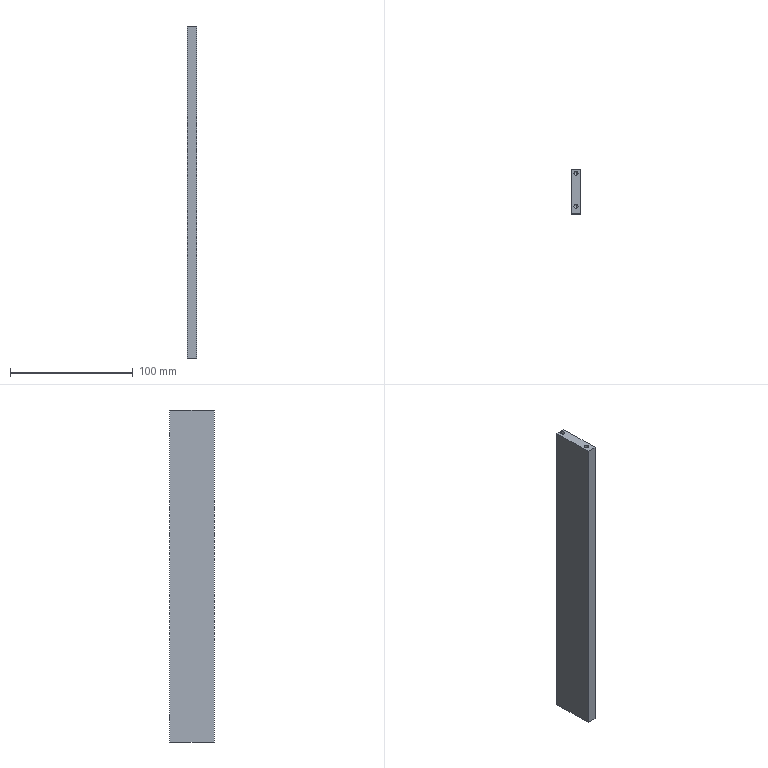Component | SolidWorks | LD101-02--Q1005-Q1-2-2 | 1 solid | 30 faces | box 8 x 36 x 270 mm | volume 77030 mm3 | cylinder 12 | cone 12 | plane 6 | commonest cylinder face diameters 3.3 x12 | material AL6061
build123d program:
from build123d import *

# Parameters (mm, degrees)
SKETCH1_W                  = 270
SKETCH1_H                  = 8
BOSS_EXTRUDE1_DEPTH        = 18
M4_TAPPED_HOLE2_AT_2_COUNT = 2
M4_TAPPED_HOLE2_AT_2_PITCH = 27
M4_TAPPED_HOLE3_D          = 3.3
M4_TAPPED_HOLE3_DEPTH      = 13.5
M4_TAPPED_HOLE3_TIP        = 0.9914


with BuildPart() as part:
    # Sketch1 → Boss-Extrude1 (new, symmetric)
    with BuildSketch(Plane.XY):
        Rectangle(SKETCH1_W, SKETCH1_H)
    extrude(amount=BOSS_EXTRUDE1_DEPTH, both=True)

    # Sketch2 → M4 Tapped Hole2 (revolve, cut)
    with BuildSketch(Plane(origin=(-135, 0, -15), x_dir=(0, 0, 1), z_dir=(0, 1, 0))):
        Polygon((0, 0), (0, 15.091), (1.65, 14.1), (1.65, 0), align=None)
    m4_tapped_hole2 = revolve(axis=Axis((-141.35, 0, -15), (1, 0, 0)), mode=Mode.SUBTRACT)

    # M4 Tapped Hole2 at 2: M4 Tapped Hole2 ×2
    with Locations(*[(0, 0, i * M4_TAPPED_HOLE2_AT_2_PITCH) for i in range(1, M4_TAPPED_HOLE2_AT_2_COUNT)]):
        add(m4_tapped_hole2, mode=Mode.SUBTRACT)

    # Mirror2: M4 Tapped Hole2 across plane
    add(m4_tapped_hole2.mirror(Plane(origin=(0, 0, 0), x_dir=(0, 0, 1), z_dir=(1, 0, 0))), mode=Mode.SUBTRACT)

    # Mirror2 copy 1 sketch → Mirror2 copy 1 (revolve, cut)
    with BuildSketch(Plane(origin=(135, 0, 12), x_dir=(0, 0, 1), z_dir=(0, 1, 0))):
        Polygon((0, 0), (0, -15.091), (1.65, -14.1), (1.65, 0), align=None)
    revolve(axis=Axis((141.35, 0, 12), (1, 0, 0)), mode=Mode.SUBTRACT)

    # M4 Tapped Hole3
    with Locations(Plane(origin=(0, 0, -18), x_dir=(-1, 0, 0), z_dir=(0, 0, -1))):
        with Locations((-115, 0), (115, 0)):
            Hole(M4_TAPPED_HOLE3_D / 2, depth=M4_TAPPED_HOLE3_DEPTH)
            with Locations((0, 0, -(M4_TAPPED_HOLE3_DEPTH + M4_TAPPED_HOLE3_TIP / 2))):  # 118° drill point
                Cone(0, M4_TAPPED_HOLE3_D / 2, M4_TAPPED_HOLE3_TIP, mode=Mode.SUBTRACT)


solid = part.part

# Placed as in the assembly
solid = solid.moved(Location((324.21, -178.897, 146.257), (90, 0, 90)))
STEP:
#1=COLOUR_RGB('',0.7922,0.8196,0.9333);
#2=FILL_AREA_STYLE_COLOUR('',#1);
#3=FILL_AREA_STYLE('',(#2));
#4=SURFACE_STYLE_FILL_AREA(#3);
#5=SURFACE_SIDE_STYLE('',(#4));
#6=SURFACE_STYLE_USAGE(.BOTH.,#5);
#7=PRESENTATION_STYLE_ASSIGNMENT((#6));
#8=CARTESIAN_POINT('',(12.764,-6.866,1.166));
#9=VERTEX_POINT('',#8);
#10=CARTESIAN_POINT('',(12.764,-6.866,1.296));
#11=VERTEX_POINT('',#10);
#12=CARTESIAN_POINT('',(12.764,-6.866,1.231));
#13=DIRECTION('',(0.,1.,0.));
#14=DIRECTION('',(0.,0.,1.));
#15=AXIS2_PLACEMENT_3D('',#12,#13,#14);
#16=CIRCLE('',#15,0.06496);
#17=EDGE_CURVE('',#9,#11,#16,.T.);
#18=ORIENTED_EDGE('',*,*,#17,.F.);
#19=CARTESIAN_POINT('',(12.764,-6.335,1.166));
#20=VERTEX_POINT('',#19);
#21=CARTESIAN_POINT('',(12.764,-6.335,1.166));
#22=DIRECTION('',(0.,1.,0.));
#23=VECTOR('',#22,39.37);
#24=LINE('',#21,#23);
#25=EDGE_CURVE('',#9,#20,#24,.T.);
#26=ORIENTED_EDGE('',*,*,#25,.T.);
#27=CARTESIAN_POINT('',(12.764,-6.335,1.296));
#28=VERTEX_POINT('',#27);
#29=CARTESIAN_POINT('',(12.764,-6.335,1.231));
#30=DIRECTION('',(0.,1.,0.));
#31=DIRECTION('',(0.,0.,1.));
#32=AXIS2_PLACEMENT_3D('',#29,#30,#31);
#33=CIRCLE('',#32,0.06496);
#34=EDGE_CURVE('',#20,#28,#33,.T.);
#35=ORIENTED_EDGE('',*,*,#34,.T.);
#36=CARTESIAN_POINT('',(12.764,-6.335,1.296));
#37=DIRECTION('',(0.,1.,0.));
#38=VECTOR('',#37,39.37);
#39=LINE('',#36,#38);
#40=EDGE_CURVE('',#11,#28,#39,.T.);
#41=ORIENTED_EDGE('',*,*,#40,.F.);
#42=EDGE_LOOP('',(#18,#26,#35,#41));
#43=FACE_OUTER_BOUND('',#42,.T.);
#44=CARTESIAN_POINT('',(12.764,-6.335,1.231));
#45=DIRECTION('',(0.,1.,0.));
#46=DIRECTION('',(0.,0.,1.));
#47=AXIS2_PLACEMENT_3D('',#44,#45,#46);
#48=CYLINDRICAL_SURFACE('',#47,0.06496);
#49=ADVANCED_FACE('',(#43),#48,.F.);
#50=CARTESIAN_POINT('',(12.764,-6.905,1.231));
#51=VERTEX_POINT('',#50);
#52=CARTESIAN_POINT('',(12.764,-6.866,1.296));
#53=DIRECTION('',(-0.,0.515,0.8572));
#54=VECTOR('',#53,39.37);
#55=LINE('',#52,#54);
#56=EDGE_CURVE('',#51,#11,#55,.T.);
#57=ORIENTED_EDGE('',*,*,#56,.F.);
#58=CARTESIAN_POINT('',(12.764,-6.866,1.166));
#59=DIRECTION('',(0.,0.515,-0.8572));
#60=VECTOR('',#59,39.37);
#61=LINE('',#58,#60);
#62=EDGE_CURVE('',#51,#9,#61,.T.);
#63=ORIENTED_EDGE('',*,*,#62,.T.);
#64=ORIENTED_EDGE('',*,*,#17,.T.);
#65=EDGE_LOOP('',(#57,#63,#64));
#66=FACE_OUTER_BOUND('',#65,.T.);
#67=CARTESIAN_POINT('',(12.764,-6.866,1.231));
#68=DIRECTION('',(0.,1.,0.));
#69=DIRECTION('',(0.,0.,1.));
#70=AXIS2_PLACEMENT_3D('',#67,#68,#69);
#71=CONICAL_SURFACE('',#70,0.06496,1.03);
#72=ADVANCED_FACE('',(#66),#71,.F.);
#73=CARTESIAN_POINT('',(12.764,-6.866,10.221));
#74=VERTEX_POINT('',#73);
#75=CARTESIAN_POINT('',(12.764,-6.866,10.351));
#76=VERTEX_POINT('',#75);
#77=CARTESIAN_POINT('',(12.764,-6.866,10.286));
#78=DIRECTION('',(0.,1.,0.));
#79=DIRECTION('',(0.,0.,1.));
#80=AXIS2_PLACEMENT_3D('',#77,#78,#79);
#81=CIRCLE('',#80,0.06496);
#82=EDGE_CURVE('',#74,#76,#81,.T.);
#83=ORIENTED_EDGE('',*,*,#82,.F.);
#84=CARTESIAN_POINT('',(12.764,-6.335,10.221));
#85=VERTEX_POINT('',#84);
#86=CARTESIAN_POINT('',(12.764,-6.335,10.221));
#87=DIRECTION('',(0.,1.,0.));
#88=VECTOR('',#87,39.37);
#89=LINE('',#86,#88);
#90=EDGE_CURVE('',#74,#85,#89,.T.);
#91=ORIENTED_EDGE('',*,*,#90,.T.);
#92=CARTESIAN_POINT('',(12.764,-6.335,10.351));
#93=VERTEX_POINT('',#92);
#94=CARTESIAN_POINT('',(12.764,-6.335,10.286));
#95=DIRECTION('',(0.,1.,0.));
#96=DIRECTION('',(0.,0.,1.));
#97=AXIS2_PLACEMENT_3D('',#94,#95,#96);
#98=CIRCLE('',#97,0.06496);
#99=EDGE_CURVE('',#85,#93,#98,.T.);
#100=ORIENTED_EDGE('',*,*,#99,.T.);
#101=CARTESIAN_POINT('',(12.764,-6.335,10.351));
#102=DIRECTION('',(0.,1.,0.));
#103=VECTOR('',#102,39.37);
#104=LINE('',#101,#103);
#105=EDGE_CURVE('',#76,#93,#104,.T.);
#106=ORIENTED_EDGE('',*,*,#105,.F.);
#107=EDGE_LOOP('',(#83,#91,#100,#106));
#108=FACE_OUTER_BOUND('',#107,.T.);
#109=CARTESIAN_POINT('',(12.764,-6.335,10.286));
#110=DIRECTION('',(0.,1.,0.));
#111=DIRECTION('',(0.,0.,1.));
#112=AXIS2_PLACEMENT_3D('',#109,#110,#111);
#113=CYLINDRICAL_SURFACE('',#112,0.06496);
#114=ADVANCED_FACE('',(#108),#113,.F.);
#115=CARTESIAN_POINT('',(12.764,-6.905,10.286));
#116=VERTEX_POINT('',#115);
#117=CARTESIAN_POINT('',(12.764,-6.866,10.351));
#118=DIRECTION('',(-0.,0.515,0.8572));
#119=VECTOR('',#118,39.37);
#120=LINE('',#117,#119);
#121=EDGE_CURVE('',#116,#76,#120,.T.);
#122=ORIENTED_EDGE('',*,*,#121,.F.);
#123=CARTESIAN_POINT('',(12.764,-6.866,10.221));
#124=DIRECTION('',(0.,0.515,-0.8572));
#125=VECTOR('',#124,39.37);
#126=LINE('',#123,#125);
#127=EDGE_CURVE('',#116,#74,#126,.T.);
#128=ORIENTED_EDGE('',*,*,#127,.T.);
#129=ORIENTED_EDGE('',*,*,#82,.T.);
#130=EDGE_LOOP('',(#122,#128,#129));
#131=FACE_OUTER_BOUND('',#130,.T.);
#132=CARTESIAN_POINT('',(12.764,-6.866,10.286));
#133=DIRECTION('',(0.,1.,0.));
#134=DIRECTION('',(0.,0.,1.));
#135=AXIS2_PLACEMENT_3D('',#132,#133,#134);
#136=CONICAL_SURFACE('',#135,0.06496,1.03);
#137=ADVANCED_FACE('',(#131),#136,.F.);
#138=CARTESIAN_POINT('',(12.764,-7.581,0.9983));
#139=VERTEX_POINT('',#138);
#140=CARTESIAN_POINT('',(12.764,-7.451,0.9983));
#141=VERTEX_POINT('',#140);
#142=CARTESIAN_POINT('',(12.764,-7.516,0.9983));
#143=DIRECTION('',(0.,0.,-1.));
#144=DIRECTION('',(0.,1.,0.));
#145=AXIS2_PLACEMENT_3D('',#142,#143,#144);
#146=CIRCLE('',#145,0.06496);
#147=EDGE_CURVE('',#139,#141,#146,.T.);
#148=ORIENTED_EDGE('',*,*,#147,.F.);
#149=CARTESIAN_POINT('',(12.764,-7.581,0.4432));
#150=VERTEX_POINT('',#149);
#151=CARTESIAN_POINT('',(12.764,-7.581,0.4432));
#152=DIRECTION('',(0.,0.,-1.));
#153=VECTOR('',#152,39.37);
#154=LINE('',#151,#153);
#155=EDGE_CURVE('',#139,#150,#154,.T.);
#156=ORIENTED_EDGE('',*,*,#155,.T.);
#157=CARTESIAN_POINT('',(12.764,-7.451,0.4432));
#158=VERTEX_POINT('',#157);
#159=CARTESIAN_POINT('',(12.764,-7.516,0.4432));
#160=DIRECTION('',(0.,0.,-1.));
#161=DIRECTION('',(0.,1.,0.));
#162=AXIS2_PLACEMENT_3D('',#159,#160,#161);
#163=CIRCLE('',#162,0.06496);
#164=EDGE_CURVE('',#150,#158,#163,.T.);
#165=ORIENTED_EDGE('',*,*,#164,.T.);
#166=CARTESIAN_POINT('',(12.764,-7.451,0.4432));
#167=DIRECTION('',(0.,0.,-1.));
#168=VECTOR('',#167,39.37);
#169=LINE('',#166,#168);
#170=EDGE_CURVE('',#141,#158,#169,.T.);
#171=ORIENTED_EDGE('',*,*,#170,.F.);
#172=EDGE_LOOP('',(#148,#156,#165,#171));
#173=FACE_OUTER_BOUND('',#172,.T.);
#174=CARTESIAN_POINT('',(12.764,-7.516,0.4432));
#175=DIRECTION('',(0.,0.,-1.));
#176=DIRECTION('',(0.,1.,0.));
#177=AXIS2_PLACEMENT_3D('',#174,#175,#176);
#178=CYLINDRICAL_SURFACE('',#177,0.06496);
#179=ADVANCED_FACE('',(#173),#178,.F.);
#180=CARTESIAN_POINT('',(12.764,-7.516,1.037));
#181=VERTEX_POINT('',#180);
#182=CARTESIAN_POINT('',(12.764,-7.451,0.9983));
#183=DIRECTION('',(0.,0.8572,-0.515));
#184=VECTOR('',#183,39.37);
#185=LINE('',#182,#184);
#186=EDGE_CURVE('',#181,#141,#185,.T.);
#187=ORIENTED_EDGE('',*,*,#186,.F.);
#188=CARTESIAN_POINT('',(12.764,-7.581,0.9983));
#189=DIRECTION('',(0.,-0.8572,-0.515));
#190=VECTOR('',#189,39.37);
#191=LINE('',#188,#190);
#192=EDGE_CURVE('',#181,#139,#191,.T.);
#193=ORIENTED_EDGE('',*,*,#192,.T.);
#194=ORIENTED_EDGE('',*,*,#147,.T.);
#195=EDGE_LOOP('',(#187,#193,#194));
#196=FACE_OUTER_BOUND('',#195,.T.);
#197=CARTESIAN_POINT('',(12.764,-7.516,0.9983));
#198=DIRECTION('',(0.,0.,-1.));
#199=DIRECTION('',(0.,1.,0.));
#200=AXIS2_PLACEMENT_3D('',#197,#198,#199);
#201=CONICAL_SURFACE('',#200,0.06496,1.03);
#202=ADVANCED_FACE('',(#196),#201,.F.);
#203=CARTESIAN_POINT('',(12.764,-6.518,0.9983));
#204=VERTEX_POINT('',#203);
#205=CARTESIAN_POINT('',(12.764,-6.388,0.9983));
#206=VERTEX_POINT('',#205);
#207=CARTESIAN_POINT('',(12.764,-6.453,0.9983));
#208=DIRECTION('',(0.,0.,-1.));
#209=DIRECTION('',(0.,1.,0.));
#210=AXIS2_PLACEMENT_3D('',#207,#208,#209);
#211=CIRCLE('',#210,0.06496);
#212=EDGE_CURVE('',#204,#206,#211,.T.);
#213=ORIENTED_EDGE('',*,*,#212,.F.);
#214=CARTESIAN_POINT('',(12.764,-6.518,0.4432));
#215=VERTEX_POINT('',#214);
#216=CARTESIAN_POINT('',(12.764,-6.518,0.4432));
#217=DIRECTION('',(0.,0.,-1.));
#218=VECTOR('',#217,39.37);
#219=LINE('',#216,#218);
#220=EDGE_CURVE('',#204,#215,#219,.T.);
#221=ORIENTED_EDGE('',*,*,#220,.T.);
#222=CARTESIAN_POINT('',(12.764,-6.388,0.4432));
#223=VERTEX_POINT('',#222);
#224=CARTESIAN_POINT('',(12.764,-6.453,0.4432));
#225=DIRECTION('',(0.,0.,-1.));
#226=DIRECTION('',(0.,1.,0.));
#227=AXIS2_PLACEMENT_3D('',#224,#225,#226);
#228=CIRCLE('',#227,0.06496);
#229=EDGE_CURVE('',#215,#223,#228,.T.);
#230=ORIENTED_EDGE('',*,*,#229,.T.);
#231=CARTESIAN_POINT('',(12.764,-6.388,0.4432));
#232=DIRECTION('',(0.,0.,-1.));
#233=VECTOR('',#232,39.37);
#234=LINE('',#231,#233);
#235=EDGE_CURVE('',#206,#223,#234,.T.);
#236=ORIENTED_EDGE('',*,*,#235,.F.);
#237=EDGE_LOOP('',(#213,#221,#230,#236));
#238=FACE_OUTER_BOUND('',#237,.T.);
#239=CARTESIAN_POINT('',(12.764,-6.453,0.4432));
#240=DIRECTION('',(0.,0.,-1.));
#241=DIRECTION('',(0.,1.,0.));
#242=AXIS2_PLACEMENT_3D('',#239,#240,#241);
#243=CYLINDRICAL_SURFACE('',#242,0.06496);
#244=ADVANCED_FACE('',(#238),#243,.F.);
#245=CARTESIAN_POINT('',(12.764,-6.453,1.037));
#246=VERTEX_POINT('',#245);
#247=CARTESIAN_POINT('',(12.764,-6.388,0.9983));
#248=DIRECTION('',(0.,0.8572,-0.515));
#249=VECTOR('',#248,39.37);
#250=LINE('',#247,#249);
#251=EDGE_CURVE('',#246,#206,#250,.T.);
#252=ORIENTED_EDGE('',*,*,#251,.F.);
#253=CARTESIAN_POINT('',(12.764,-6.518,0.9983));
#254=DIRECTION('',(0.,-0.8572,-0.515));
#255=VECTOR('',#254,39.37);
#256=LINE('',#253,#255);
#257=EDGE_CURVE('',#246,#204,#256,.T.);
#258=ORIENTED_EDGE('',*,*,#257,.T.);
#259=ORIENTED_EDGE('',*,*,#212,.T.);
#260=EDGE_LOOP('',(#252,#258,#259));
#261=FACE_OUTER_BOUND('',#260,.T.);
#262=CARTESIAN_POINT('',(12.764,-6.453,0.9983));
#263=DIRECTION('',(0.,0.,-1.));
#264=DIRECTION('',(0.,1.,0.));
#265=AXIS2_PLACEMENT_3D('',#262,#263,#264);
#266=CONICAL_SURFACE('',#265,0.06496,1.03);
#267=ADVANCED_FACE('',(#261),#266,.F.);
#268=CARTESIAN_POINT('',(12.764,-7.451,10.518));
#269=VERTEX_POINT('',#268);
#270=CARTESIAN_POINT('',(12.764,-7.581,10.518));
#271=VERTEX_POINT('',#270);
#272=CARTESIAN_POINT('',(12.764,-7.516,10.518));
#273=DIRECTION('',(-0.,0.,1.));
#274=DIRECTION('',(0.,-1.,0.));
#275=AXIS2_PLACEMENT_3D('',#272,#273,#274);
#276=CIRCLE('',#275,0.06496);
#277=EDGE_CURVE('',#269,#271,#276,.T.);
#278=ORIENTED_EDGE('',*,*,#277,.F.);
#279=CARTESIAN_POINT('',(12.764,-7.451,11.073));
#280=VERTEX_POINT('',#279);
#281=CARTESIAN_POINT('',(12.764,-7.451,11.073));
#282=DIRECTION('',(-0.,0.,1.));
#283=VECTOR('',#282,39.37);
#284=LINE('',#281,#283);
#285=EDGE_CURVE('',#269,#280,#284,.T.);
#286=ORIENTED_EDGE('',*,*,#285,.T.);
#287=CARTESIAN_POINT('',(12.764,-7.581,11.073));
#288=VERTEX_POINT('',#287);
#289=CARTESIAN_POINT('',(12.764,-7.516,11.073));
#290=DIRECTION('',(-0.,0.,1.));
#291=DIRECTION('',(0.,-1.,0.));
#292=AXIS2_PLACEMENT_3D('',#289,#290,#291);
#293=CIRCLE('',#292,0.06496);
#294=EDGE_CURVE('',#280,#288,#293,.T.);
#295=ORIENTED_EDGE('',*,*,#294,.T.);
#296=CARTESIAN_POINT('',(12.764,-7.581,11.073));
#297=DIRECTION('',(-0.,0.,1.));
#298=VECTOR('',#297,39.37);
#299=LINE('',#296,#298);
#300=EDGE_CURVE('',#271,#288,#299,.T.);
#301=ORIENTED_EDGE('',*,*,#300,.F.);
#302=EDGE_LOOP('',(#278,#286,#295,#301));
#303=FACE_OUTER_BOUND('',#302,.T.);
#304=CARTESIAN_POINT('',(12.764,-7.516,11.073));
#305=DIRECTION('',(-0.,0.,1.));
#306=DIRECTION('',(0.,-1.,0.));
#307=AXIS2_PLACEMENT_3D('',#304,#305,#306);
#308=CYLINDRICAL_SURFACE('',#307,0.06496);
#309=ADVANCED_FACE('',(#303),#308,.F.);
#310=CARTESIAN_POINT('',(12.764,-7.516,10.479));
#311=VERTEX_POINT('',#310);
#312=CARTESIAN_POINT('',(12.764,-7.581,10.518));
#313=DIRECTION('',(-0.,-0.8572,0.515));
#314=VECTOR('',#313,39.37);
#315=LINE('',#312,#314);
#316=EDGE_CURVE('',#311,#271,#315,.T.);
#317=ORIENTED_EDGE('',*,*,#316,.F.);
#318=CARTESIAN_POINT('',(12.764,-7.451,10.518));
#319=DIRECTION('',(0.,0.8572,0.515));
#320=VECTOR('',#319,39.37);
#321=LINE('',#318,#320);
#322=EDGE_CURVE('',#311,#269,#321,.T.);
#323=ORIENTED_EDGE('',*,*,#322,.T.);
#324=ORIENTED_EDGE('',*,*,#277,.T.);
#325=EDGE_LOOP('',(#317,#323,#324));
#326=FACE_OUTER_BOUND('',#325,.T.);
#327=CARTESIAN_POINT('',(12.764,-7.516,10.518));
#328=DIRECTION('',(-0.,0.,1.));
#329=DIRECTION('',(0.,-1.,0.));
#330=AXIS2_PLACEMENT_3D('',#327,#328,#329);
#331=CONICAL_SURFACE('',#330,0.06496,1.03);
#332=ADVANCED_FACE('',(#326),#331,.F.);
#333=CARTESIAN_POINT('',(12.764,-6.388,10.518));
#334=VERTEX_POINT('',#333);
#335=CARTESIAN_POINT('',(12.764,-6.518,10.518));
#336=VERTEX_POINT('',#335);
#337=CARTESIAN_POINT('',(12.764,-6.453,10.518));
#338=DIRECTION('',(-0.,0.,1.));
#339=DIRECTION('',(0.,-1.,0.));
#340=AXIS2_PLACEMENT_3D('',#337,#338,#339);
#341=CIRCLE('',#340,0.06496);
#342=EDGE_CURVE('',#334,#336,#341,.T.);
#343=ORIENTED_EDGE('',*,*,#342,.F.);
#344=CARTESIAN_POINT('',(12.764,-6.388,11.073));
#345=VERTEX_POINT('',#344);
#346=CARTESIAN_POINT('',(12.764,-6.388,11.073));
#347=DIRECTION('',(-0.,0.,1.));
#348=VECTOR('',#347,39.37);
#349=LINE('',#346,#348);
#350=EDGE_CURVE('',#334,#345,#349,.T.);
#351=ORIENTED_EDGE('',*,*,#350,.T.);
#352=CARTESIAN_POINT('',(12.764,-6.518,11.073));
#353=VERTEX_POINT('',#352);
#354=CARTESIAN_POINT('',(12.764,-6.453,11.073));
#355=DIRECTION('',(-0.,0.,1.));
#356=DIRECTION('',(0.,-1.,0.));
#357=AXIS2_PLACEMENT_3D('',#354,#355,#356);
#358=CIRCLE('',#357,0.06496);
#359=EDGE_CURVE('',#345,#353,#358,.T.);
#360=ORIENTED_EDGE('',*,*,#359,.T.);
#361=CARTESIAN_POINT('',(12.764,-6.518,11.073));
#362=DIRECTION('',(-0.,0.,1.));
#363=VECTOR('',#362,39.37);
#364=LINE('',#361,#363);
#365=EDGE_CURVE('',#336,#353,#364,.T.);
#366=ORIENTED_EDGE('',*,*,#365,.F.);
#367=EDGE_LOOP('',(#343,#351,#360,#366));
#368=FACE_OUTER_BOUND('',#367,.T.);
#369=CARTESIAN_POINT('',(12.764,-6.453,11.073));
#370=DIRECTION('',(-0.,0.,1.));
#371=DIRECTION('',(0.,-1.,0.));
#372=AXIS2_PLACEMENT_3D('',#369,#370,#371);
#373=CYLINDRICAL_SURFACE('',#372,0.06496);
#374=ADVANCED_FACE('',(#368),#373,.F.);
#375=CARTESIAN_POINT('',(12.764,-6.453,10.479));
#376=VERTEX_POINT('',#375);
#377=CARTESIAN_POINT('',(12.764,-6.518,10.518));
#378=DIRECTION('',(-0.,-0.8572,0.515));
#379=VECTOR('',#378,39.37);
#380=LINE('',#377,#379);
#381=EDGE_CURVE('',#376,#336,#380,.T.);
#382=ORIENTED_EDGE('',*,*,#381,.F.);
#383=CARTESIAN_POINT('',(12.764,-6.388,10.518));
#384=DIRECTION('',(0.,0.8572,0.515));
#385=VECTOR('',#384,39.37);
#386=LINE('',#383,#385);
#387=EDGE_CURVE('',#376,#334,#386,.T.);
#388=ORIENTED_EDGE('',*,*,#387,.T.);
#389=ORIENTED_EDGE('',*,*,#342,.T.);
#390=EDGE_LOOP('',(#382,#388,#389));
#391=FACE_OUTER_BOUND('',#390,.T.);
#392=CARTESIAN_POINT('',(12.764,-6.453,10.518));
#393=DIRECTION('',(-0.,0.,1.));
#394=DIRECTION('',(0.,-1.,0.));
#395=AXIS2_PLACEMENT_3D('',#392,#393,#394);
#396=CONICAL_SURFACE('',#395,0.06496,1.03);
#397=ADVANCED_FACE('',(#391),#396,.F.);
#398=CARTESIAN_POINT('',(12.764,-7.516,0.4432));
#399=DIRECTION('',(0.,0.,-1.));
#400=DIRECTION('',(0.,1.,0.));
#401=AXIS2_PLACEMENT_3D('',#398,#399,#400);
#402=CIRCLE('',#401,0.06496);
#403=EDGE_CURVE('',#158,#150,#402,.T.);
#404=ORIENTED_EDGE('',*,*,#403,.F.);
#405=ORIENTED_EDGE('',*,*,#164,.F.);
#406=EDGE_LOOP('',(#404,#405));
#407=FACE_BOUND('',#406,.T.);
#408=CARTESIAN_POINT('',(12.764,-6.453,0.4432));
#409=DIRECTION('',(0.,0.,-1.));
#410=DIRECTION('',(0.,1.,0.));
#411=AXIS2_PLACEMENT_3D('',#408,#409,#410);
#412=CIRCLE('',#411,0.06496);
#413=EDGE_CURVE('',#223,#215,#412,.T.);
#414=ORIENTED_EDGE('',*,*,#413,.F.);
#415=ORIENTED_EDGE('',*,*,#229,.F.);
#416=EDGE_LOOP('',(#414,#415));
#417=FACE_BOUND('',#416,.T.);
#418=CARTESIAN_POINT('',(12.607,-6.335,0.4432));
#419=VERTEX_POINT('',#418);
#420=CARTESIAN_POINT('',(12.922,-6.335,0.4432));
#421=VERTEX_POINT('',#420);
#422=CARTESIAN_POINT('',(12.607,-6.335,0.4432));
#423=DIRECTION('',(1.,0.,0.));
#424=VECTOR('',#423,39.37);
#425=LINE('',#422,#424);
#426=EDGE_CURVE('',#419,#421,#425,.T.);
#427=ORIENTED_EDGE('',*,*,#426,.T.);
#428=CARTESIAN_POINT('',(12.922,-7.752,0.4432));
#429=VERTEX_POINT('',#428);
#430=CARTESIAN_POINT('',(12.922,-7.752,0.4432));
#431=DIRECTION('',(0.,1.,0.));
#432=VECTOR('',#431,39.37);
#433=LINE('',#430,#432);
#434=EDGE_CURVE('',#429,#421,#433,.T.);
#435=ORIENTED_EDGE('',*,*,#434,.F.);
#436=CARTESIAN_POINT('',(12.607,-7.752,0.4432));
#437=VERTEX_POINT('',#436);
#438=CARTESIAN_POINT('',(12.607,-7.752,0.4432));
#439=DIRECTION('',(1.,0.,0.));
#440=VECTOR('',#439,39.37);
#441=LINE('',#438,#440);
#442=EDGE_CURVE('',#437,#429,#441,.T.);
#443=ORIENTED_EDGE('',*,*,#442,.F.);
#444=CARTESIAN_POINT('',(12.607,-7.752,0.4432));
#445=DIRECTION('',(0.,1.,0.));
#446=VECTOR('',#445,39.37);
#447=LINE('',#444,#446);
#448=EDGE_CURVE('',#437,#419,#447,.T.);
#449=ORIENTED_EDGE('',*,*,#448,.T.);
#450=EDGE_LOOP('',(#427,#435,#443,#449));
#451=FACE_OUTER_BOUND('',#450,.T.);
#452=CARTESIAN_POINT('',(12.607,-7.752,0.4432));
#453=DIRECTION('',(-0.,0.,1.));
#454=DIRECTION('',(0.,-1.,0.));
#455=AXIS2_PLACEMENT_3D('',#452,#453,#454);
#456=PLANE('',#455);
#457=ADVANCED_FACE('',(#407,#417,#451),#456,.F.);
#458=CARTESIAN_POINT('',(12.922,-6.335,11.073));
#459=VERTEX_POINT('',#458);
#460=CARTESIAN_POINT('',(12.922,-6.335,11.073));
#461=DIRECTION('',(-0.,0.,1.));
#462=VECTOR('',#461,39.37);
#463=LINE('',#460,#462);
#464=EDGE_CURVE('',#421,#459,#463,.T.);
#465=ORIENTED_EDGE('',*,*,#464,.T.);
#466=CARTESIAN_POINT('',(12.922,-7.752,11.073));
#467=VERTEX_POINT('',#466);
#468=CARTESIAN_POINT('',(12.922,-7.752,11.073));
#469=DIRECTION('',(0.,1.,0.));
#470=VECTOR('',#469,39.37);
#471=LINE('',#468,#470);
#472=EDGE_CURVE('',#467,#459,#471,.T.);
#473=ORIENTED_EDGE('',*,*,#472,.F.);
#474=CARTESIAN_POINT('',(12.922,-7.752,11.073));
#475=DIRECTION('',(-0.,0.,1.));
#476=VECTOR('',#475,39.37);
#477=LINE('',#474,#476);
#478=EDGE_CURVE('',#429,#467,#477,.T.);
#479=ORIENTED_EDGE('',*,*,#478,.F.);
#480=ORIENTED_EDGE('',*,*,#434,.T.);
#481=EDGE_LOOP('',(#465,#473,#479,#480));
#482=FACE_OUTER_BOUND('',#481,.T.);
#483=CARTESIAN_POINT('',(12.922,-7.752,11.073));
#484=DIRECTION('',(-1.,0.,-0.));
#485=DIRECTION('',(0.,1.,0.));
#486=AXIS2_PLACEMENT_3D('',#483,#484,#485);
#487=PLANE('',#486);
#488=ADVANCED_FACE('',(#482),#487,.F.);
#489=CARTESIAN_POINT('',(12.764,-7.516,11.073));
#490=DIRECTION('',(-0.,0.,1.));
#491=DIRECTION('',(0.,-1.,0.));
#492=AXIS2_PLACEMENT_3D('',#489,#490,#491);
#493=CIRCLE('',#492,0.06496);
#494=EDGE_CURVE('',#288,#280,#493,.T.);
#495=ORIENTED_EDGE('',*,*,#494,.F.);
#496=ORIENTED_EDGE('',*,*,#294,.F.);
#497=EDGE_LOOP('',(#495,#496));
#498=FACE_BOUND('',#497,.T.);
#499=CARTESIAN_POINT('',(12.764,-6.453,11.073));
#500=DIRECTION('',(-0.,0.,1.));
#501=DIRECTION('',(0.,-1.,0.));
#502=AXIS2_PLACEMENT_3D('',#499,#500,#501);
#503=CIRCLE('',#502,0.06496);
#504=EDGE_CURVE('',#353,#345,#503,.T.);
#505=ORIENTED_EDGE('',*,*,#504,.F.);
#506=ORIENTED_EDGE('',*,*,#359,.F.);
#507=EDGE_LOOP('',(#505,#506));
#508=FACE_BOUND('',#507,.T.);
#509=CARTESIAN_POINT('',(12.607,-6.335,11.073));
#510=VERTEX_POINT('',#509);
#511=CARTESIAN_POINT('',(12.607,-6.335,11.073));
#512=DIRECTION('',(-1.,0.,-0.));
#513=VECTOR('',#512,39.37);
#514=LINE('',#511,#513);
#515=EDGE_CURVE('',#459,#510,#514,.T.);
#516=ORIENTED_EDGE('',*,*,#515,.T.);
#517=CARTESIAN_POINT('',(12.607,-7.752,11.073));
#518=VERTEX_POINT('',#517);
#519=CARTESIAN_POINT('',(12.607,-7.752,11.073));
#520=DIRECTION('',(0.,1.,0.));
#521=VECTOR('',#520,39.37);
#522=LINE('',#519,#521);
#523=EDGE_CURVE('',#518,#510,#522,.T.);
#524=ORIENTED_EDGE('',*,*,#523,.F.);
#525=CARTESIAN_POINT('',(12.607,-7.752,11.073));
#526=DIRECTION('',(-1.,0.,-0.));
#527=VECTOR('',#526,39.37);
#528=LINE('',#525,#527);
#529=EDGE_CURVE('',#467,#518,#528,.T.);
#530=ORIENTED_EDGE('',*,*,#529,.F.);
#531=ORIENTED_EDGE('',*,*,#472,.T.);
#532=EDGE_LOOP('',(#516,#524,#530,#531));
#533=FACE_OUTER_BOUND('',#532,.T.);
#534=CARTESIAN_POINT('',(12.607,-7.752,11.073));
#535=DIRECTION('',(0.,0.,-1.));
#536=DIRECTION('',(0.,1.,0.));
#537=AXIS2_PLACEMENT_3D('',#534,#535,#536);
#538=PLANE('',#537);
#539=ADVANCED_FACE('',(#498,#508,#533),#538,.F.);
#540=CARTESIAN_POINT('',(12.607,-6.335,11.073));
#541=DIRECTION('',(0.,0.,-1.));
#542=VECTOR('',#541,39.37);
#543=LINE('',#540,#542);
#544=EDGE_CURVE('',#510,#419,#543,.T.);
#545=ORIENTED_EDGE('',*,*,#544,.T.);
#546=ORIENTED_EDGE('',*,*,#448,.F.);
#547=CARTESIAN_POINT('',(12.607,-7.752,11.073));
#548=DIRECTION('',(0.,0.,-1.));
#549=VECTOR('',#548,39.37);
#550=LINE('',#547,#549);
#551=EDGE_CURVE('',#518,#437,#550,.T.);
#552=ORIENTED_EDGE('',*,*,#551,.F.);
#553=ORIENTED_EDGE('',*,*,#523,.T.);
#554=EDGE_LOOP('',(#545,#546,#552,#553));
#555=FACE_OUTER_BOUND('',#554,.T.);
#556=CARTESIAN_POINT('',(12.607,-7.752,11.073));
#557=DIRECTION('',(1.,0.,0.));
#558=DIRECTION('',(0.,-1.,0.));
#559=AXIS2_PLACEMENT_3D('',#556,#557,#558);
#560=PLANE('',#559);
#561=ADVANCED_FACE('',(#555),#560,.F.);
#562=ORIENTED_EDGE('',*,*,#442,.T.);
#563=ORIENTED_EDGE('',*,*,#478,.T.);
#564=ORIENTED_EDGE('',*,*,#529,.T.);
#565=ORIENTED_EDGE('',*,*,#551,.T.);
#566=EDGE_LOOP('',(#562,#563,#564,#565));
#567=FACE_OUTER_BOUND('',#566,.T.);
#568=CARTESIAN_POINT('',(12.764,-7.752,5.758));
#569=DIRECTION('',(0.,1.,0.));
#570=DIRECTION('',(-0.,0.,1.));
#571=AXIS2_PLACEMENT_3D('',#568,#569,#570);
#572=PLANE('',#571);
#573=ADVANCED_FACE('',(#567),#572,.F.);
#574=CARTESIAN_POINT('',(12.764,-6.335,1.231));
#575=DIRECTION('',(0.,1.,0.));
#576=DIRECTION('',(0.,0.,1.));
#577=AXIS2_PLACEMENT_3D('',#574,#575,#576);
#578=CIRCLE('',#577,0.06496);
#579=EDGE_CURVE('',#28,#20,#578,.T.);
#580=ORIENTED_EDGE('',*,*,#579,.F.);
#581=ORIENTED_EDGE('',*,*,#34,.F.);
#582=EDGE_LOOP('',(#580,#581));
#583=FACE_BOUND('',#582,.T.);
#584=CARTESIAN_POINT('',(12.764,-6.335,10.286));
#585=DIRECTION('',(0.,1.,0.));
#586=DIRECTION('',(0.,0.,1.));
#587=AXIS2_PLACEMENT_3D('',#584,#585,#586);
#588=CIRCLE('',#587,0.06496);
#589=EDGE_CURVE('',#93,#85,#588,.T.);
#590=ORIENTED_EDGE('',*,*,#589,.F.);
#591=ORIENTED_EDGE('',*,*,#99,.F.);
#592=EDGE_LOOP('',(#590,#591));
#593=FACE_BOUND('',#592,.T.);
#594=ORIENTED_EDGE('',*,*,#426,.F.);
#595=ORIENTED_EDGE('',*,*,#544,.F.);
#596=ORIENTED_EDGE('',*,*,#515,.F.);
#597=ORIENTED_EDGE('',*,*,#464,.F.);
#598=EDGE_LOOP('',(#594,#595,#596,#597));
#599=FACE_OUTER_BOUND('',#598,.T.);
#600=CARTESIAN_POINT('',(12.764,-6.335,5.758));
#601=DIRECTION('',(0.,1.,0.));
#602=DIRECTION('',(-0.,0.,1.));
#603=AXIS2_PLACEMENT_3D('',#600,#601,#602);
#604=PLANE('',#603);
#605=ADVANCED_FACE('',(#583,#593,#599),#604,.T.);
#606=ORIENTED_EDGE('',*,*,#387,.F.);
#607=ORIENTED_EDGE('',*,*,#381,.T.);
#608=CARTESIAN_POINT('',(12.764,-6.453,10.518));
#609=DIRECTION('',(-0.,0.,1.));
#610=DIRECTION('',(0.,-1.,0.));
#611=AXIS2_PLACEMENT_3D('',#608,#609,#610);
#612=CIRCLE('',#611,0.06496);
#613=EDGE_CURVE('',#336,#334,#612,.T.);
#614=ORIENTED_EDGE('',*,*,#613,.T.);
#615=EDGE_LOOP('',(#606,#607,#614));
#616=FACE_OUTER_BOUND('',#615,.T.);
#617=CARTESIAN_POINT('',(12.764,-6.453,10.518));
#618=DIRECTION('',(-0.,0.,1.));
#619=DIRECTION('',(0.,-1.,0.));
#620=AXIS2_PLACEMENT_3D('',#617,#618,#619);
#621=CONICAL_SURFACE('',#620,0.06496,1.03);
#622=ADVANCED_FACE('',(#616),#621,.F.);
#623=ORIENTED_EDGE('',*,*,#350,.F.);
#624=ORIENTED_EDGE('',*,*,#613,.F.);
#625=ORIENTED_EDGE('',*,*,#365,.T.);
#626=ORIENTED_EDGE('',*,*,#504,.T.);
#627=EDGE_LOOP('',(#623,#624,#625,#626));
#628=FACE_OUTER_BOUND('',#627,.T.);
#629=CARTESIAN_POINT('',(12.764,-6.453,11.073));
#630=DIRECTION('',(-0.,0.,1.));
#631=DIRECTION('',(0.,-1.,0.));
#632=AXIS2_PLACEMENT_3D('',#629,#630,#631);
#633=CYLINDRICAL_SURFACE('',#632,0.06496);
#634=ADVANCED_FACE('',(#628),#633,.F.);
#635=ORIENTED_EDGE('',*,*,#322,.F.);
#636=ORIENTED_EDGE('',*,*,#316,.T.);
#637=CARTESIAN_POINT('',(12.764,-7.516,10.518));
#638=DIRECTION('',(-0.,0.,1.));
#639=DIRECTION('',(0.,-1.,0.));
#640=AXIS2_PLACEMENT_3D('',#637,#638,#639);
#641=CIRCLE('',#640,0.06496);
#642=EDGE_CURVE('',#271,#269,#641,.T.);
#643=ORIENTED_EDGE('',*,*,#642,.T.);
#644=EDGE_LOOP('',(#635,#636,#643));
#645=FACE_OUTER_BOUND('',#644,.T.);
#646=CARTESIAN_POINT('',(12.764,-7.516,10.518));
#647=DIRECTION('',(-0.,0.,1.));
#648=DIRECTION('',(0.,-1.,0.));
#649=AXIS2_PLACEMENT_3D('',#646,#647,#648);
#650=CONICAL_SURFACE('',#649,0.06496,1.03);
#651=ADVANCED_FACE('',(#645),#650,.F.);
#652=ORIENTED_EDGE('',*,*,#285,.F.);
#653=ORIENTED_EDGE('',*,*,#642,.F.);
#654=ORIENTED_EDGE('',*,*,#300,.T.);
#655=ORIENTED_EDGE('',*,*,#494,.T.);
#656=EDGE_LOOP('',(#652,#653,#654,#655));
#657=FACE_OUTER_BOUND('',#656,.T.);
#658=CARTESIAN_POINT('',(12.764,-7.516,11.073));
#659=DIRECTION('',(-0.,0.,1.));
#660=DIRECTION('',(0.,-1.,0.));
#661=AXIS2_PLACEMENT_3D('',#658,#659,#660);
#662=CYLINDRICAL_SURFACE('',#661,0.06496);
#663=ADVANCED_FACE('',(#657),#662,.F.);
#664=ORIENTED_EDGE('',*,*,#257,.F.);
#665=ORIENTED_EDGE('',*,*,#251,.T.);
#666=CARTESIAN_POINT('',(12.764,-6.453,0.9983));
#667=DIRECTION('',(0.,0.,-1.));
#668=DIRECTION('',(0.,1.,0.));
#669=AXIS2_PLACEMENT_3D('',#666,#667,#668);
#670=CIRCLE('',#669,0.06496);
#671=EDGE_CURVE('',#206,#204,#670,.T.);
#672=ORIENTED_EDGE('',*,*,#671,.T.);
#673=EDGE_LOOP('',(#664,#665,#672));
#674=FACE_OUTER_BOUND('',#673,.T.);
#675=CARTESIAN_POINT('',(12.764,-6.453,0.9983));
#676=DIRECTION('',(0.,0.,-1.));
#677=DIRECTION('',(0.,1.,0.));
#678=AXIS2_PLACEMENT_3D('',#675,#676,#677);
#679=CONICAL_SURFACE('',#678,0.06496,1.03);
#680=ADVANCED_FACE('',(#674),#679,.F.);
#681=ORIENTED_EDGE('',*,*,#220,.F.);
#682=ORIENTED_EDGE('',*,*,#671,.F.);
#683=ORIENTED_EDGE('',*,*,#235,.T.);
#684=ORIENTED_EDGE('',*,*,#413,.T.);
#685=EDGE_LOOP('',(#681,#682,#683,#684));
#686=FACE_OUTER_BOUND('',#685,.T.);
#687=CARTESIAN_POINT('',(12.764,-6.453,0.4432));
#688=DIRECTION('',(0.,0.,-1.));
#689=DIRECTION('',(0.,1.,0.));
#690=AXIS2_PLACEMENT_3D('',#687,#688,#689);
#691=CYLINDRICAL_SURFACE('',#690,0.06496);
#692=ADVANCED_FACE('',(#686),#691,.F.);
#693=ORIENTED_EDGE('',*,*,#192,.F.);
#694=ORIENTED_EDGE('',*,*,#186,.T.);
#695=CARTESIAN_POINT('',(12.764,-7.516,0.9983));
#696=DIRECTION('',(0.,0.,-1.));
#697=DIRECTION('',(0.,1.,0.));
#698=AXIS2_PLACEMENT_3D('',#695,#696,#697);
#699=CIRCLE('',#698,0.06496);
#700=EDGE_CURVE('',#141,#139,#699,.T.);
#701=ORIENTED_EDGE('',*,*,#700,.T.);
#702=EDGE_LOOP('',(#693,#694,#701));
#703=FACE_OUTER_BOUND('',#702,.T.);
#704=CARTESIAN_POINT('',(12.764,-7.516,0.9983));
#705=DIRECTION('',(0.,0.,-1.));
#706=DIRECTION('',(0.,1.,0.));
#707=AXIS2_PLACEMENT_3D('',#704,#705,#706);
#708=CONICAL_SURFACE('',#707,0.06496,1.03);
#709=ADVANCED_FACE('',(#703),#708,.F.);
#710=ORIENTED_EDGE('',*,*,#155,.F.);
#711=ORIENTED_EDGE('',*,*,#700,.F.);
#712=ORIENTED_EDGE('',*,*,#170,.T.);
#713=ORIENTED_EDGE('',*,*,#403,.T.);
#714=EDGE_LOOP('',(#710,#711,#712,#713));
#715=FACE_OUTER_BOUND('',#714,.T.);
#716=CARTESIAN_POINT('',(12.764,-7.516,0.4432));
#717=DIRECTION('',(0.,0.,-1.));
#718=DIRECTION('',(0.,1.,0.));
#719=AXIS2_PLACEMENT_3D('',#716,#717,#718);
#720=CYLINDRICAL_SURFACE('',#719,0.06496);
#721=ADVANCED_FACE('',(#715),#720,.F.);
#722=ORIENTED_EDGE('',*,*,#127,.F.);
#723=ORIENTED_EDGE('',*,*,#121,.T.);
#724=CARTESIAN_POINT('',(12.764,-6.866,10.286));
#725=DIRECTION('',(0.,1.,0.));
#726=DIRECTION('',(0.,0.,1.));
#727=AXIS2_PLACEMENT_3D('',#724,#725,#726);
#728=CIRCLE('',#727,0.06496);
#729=EDGE_CURVE('',#76,#74,#728,.T.);
#730=ORIENTED_EDGE('',*,*,#729,.T.);
#731=EDGE_LOOP('',(#722,#723,#730));
#732=FACE_OUTER_BOUND('',#731,.T.);
#733=CARTESIAN_POINT('',(12.764,-6.866,10.286));
#734=DIRECTION('',(0.,1.,0.));
#735=DIRECTION('',(0.,0.,1.));
#736=AXIS2_PLACEMENT_3D('',#733,#734,#735);
#737=CONICAL_SURFACE('',#736,0.06496,1.03);
#738=ADVANCED_FACE('',(#732),#737,.F.);
#739=ORIENTED_EDGE('',*,*,#90,.F.);
#740=ORIENTED_EDGE('',*,*,#729,.F.);
#741=ORIENTED_EDGE('',*,*,#105,.T.);
#742=ORIENTED_EDGE('',*,*,#589,.T.);
#743=EDGE_LOOP('',(#739,#740,#741,#742));
#744=FACE_OUTER_BOUND('',#743,.T.);
#745=CARTESIAN_POINT('',(12.764,-6.335,10.286));
#746=DIRECTION('',(0.,1.,0.));
#747=DIRECTION('',(0.,0.,1.));
#748=AXIS2_PLACEMENT_3D('',#745,#746,#747);
#749=CYLINDRICAL_SURFACE('',#748,0.06496);
#750=ADVANCED_FACE('',(#744),#749,.F.);
#751=ORIENTED_EDGE('',*,*,#62,.F.);
#752=ORIENTED_EDGE('',*,*,#56,.T.);
#753=CARTESIAN_POINT('',(12.764,-6.866,1.231));
#754=DIRECTION('',(0.,1.,0.));
#755=DIRECTION('',(0.,0.,1.));
#756=AXIS2_PLACEMENT_3D('',#753,#754,#755);
#757=CIRCLE('',#756,0.06496);
#758=EDGE_CURVE('',#11,#9,#757,.T.);
#759=ORIENTED_EDGE('',*,*,#758,.T.);
#760=EDGE_LOOP('',(#751,#752,#759));
#761=FACE_OUTER_BOUND('',#760,.T.);
#762=CARTESIAN_POINT('',(12.764,-6.866,1.231));
#763=DIRECTION('',(0.,1.,0.));
#764=DIRECTION('',(0.,0.,1.));
#765=AXIS2_PLACEMENT_3D('',#762,#763,#764);
#766=CONICAL_SURFACE('',#765,0.06496,1.03);
#767=ADVANCED_FACE('',(#761),#766,.F.);
#768=ORIENTED_EDGE('',*,*,#25,.F.);
#769=ORIENTED_EDGE('',*,*,#758,.F.);
#770=ORIENTED_EDGE('',*,*,#40,.T.);
#771=ORIENTED_EDGE('',*,*,#579,.T.);
#772=EDGE_LOOP('',(#768,#769,#770,#771));
#773=FACE_OUTER_BOUND('',#772,.T.);
#774=CARTESIAN_POINT('',(12.764,-6.335,1.231));
#775=DIRECTION('',(0.,1.,0.));
#776=DIRECTION('',(0.,0.,1.));
#777=AXIS2_PLACEMENT_3D('',#774,#775,#776);
#778=CYLINDRICAL_SURFACE('',#777,0.06496);
#779=ADVANCED_FACE('',(#773),#778,.F.);
#780=CLOSED_SHELL('',(#49,#72,#114,#137,#179,#202,#244,#267,#309,#332,#374,#397,#457,#488,#539,#561,#573,#605,#622,#634,#651,#663,#680,#692,#709,#721,#738,#750,#767,#779));
#781=MANIFOLD_SOLID_BREP('',#780);
#782=STYLED_ITEM('',(#7),#781);
#783=(LENGTH_UNIT()NAMED_UNIT(*)SI_UNIT($,.METRE.));
#784=LENGTH_MEASURE_WITH_UNIT(LENGTH_MEASURE(0.0254),#783);
#785=DIMENSIONAL_EXPONENTS(1.,0.,0.,0.,0.,0.,0.);
#786=(CONVERSION_BASED_UNIT('',#784)LENGTH_UNIT()NAMED_UNIT(#785));
#787=UNCERTAINTY_MEASURE_WITH_UNIT(LENGTH_MEASURE(0.00001),#786,'','');
#788=(NAMED_UNIT(*)PLANE_ANGLE_UNIT()SI_UNIT($,.RADIAN.));
#789=(NAMED_UNIT(*)SI_UNIT($,.STERADIAN.)SOLID_ANGLE_UNIT());
#790=(GEOMETRIC_REPRESENTATION_CONTEXT(3)GLOBAL_UNCERTAINTY_ASSIGNED_CONTEXT((#787))GLOBAL_UNIT_ASSIGNED_CONTEXT((#786,#788,#789))REPRESENTATION_CONTEXT('',''));
#791=MECHANICAL_DESIGN_GEOMETRIC_PRESENTATION_REPRESENTATION('',(#782),#790);
#792=CARTESIAN_POINT('',(0.,0.,0.));
#793=DIRECTION('',(0.,0.,1.));
#794=DIRECTION('',(1.,0.,0.));
#795=AXIS2_PLACEMENT_3D('',#792,#793,#794);
#796=(LENGTH_UNIT()NAMED_UNIT(*)SI_UNIT($,.METRE.));
#797=LENGTH_MEASURE_WITH_UNIT(LENGTH_MEASURE(0.0254),#796);
#798=DIMENSIONAL_EXPONENTS(1.,0.,0.,0.,0.,0.,0.);
#799=(CONVERSION_BASED_UNIT('',#797)LENGTH_UNIT()NAMED_UNIT(#798));
#800=UNCERTAINTY_MEASURE_WITH_UNIT(LENGTH_MEASURE(0.00001),#799,'','');
#801=(NAMED_UNIT(*)PLANE_ANGLE_UNIT()SI_UNIT($,.RADIAN.));
#802=(NAMED_UNIT(*)SI_UNIT($,.STERADIAN.)SOLID_ANGLE_UNIT());
#803=(GEOMETRIC_REPRESENTATION_CONTEXT(3)GLOBAL_UNCERTAINTY_ASSIGNED_CONTEXT((#800))GLOBAL_UNIT_ASSIGNED_CONTEXT((#799,#801,#802))REPRESENTATION_CONTEXT('',''));
#804=ADVANCED_BREP_SHAPE_REPRESENTATION('',(#781,#795),#803);
#805=PRESENTATION_LAYER_ASSIGNMENT('','',(#782));